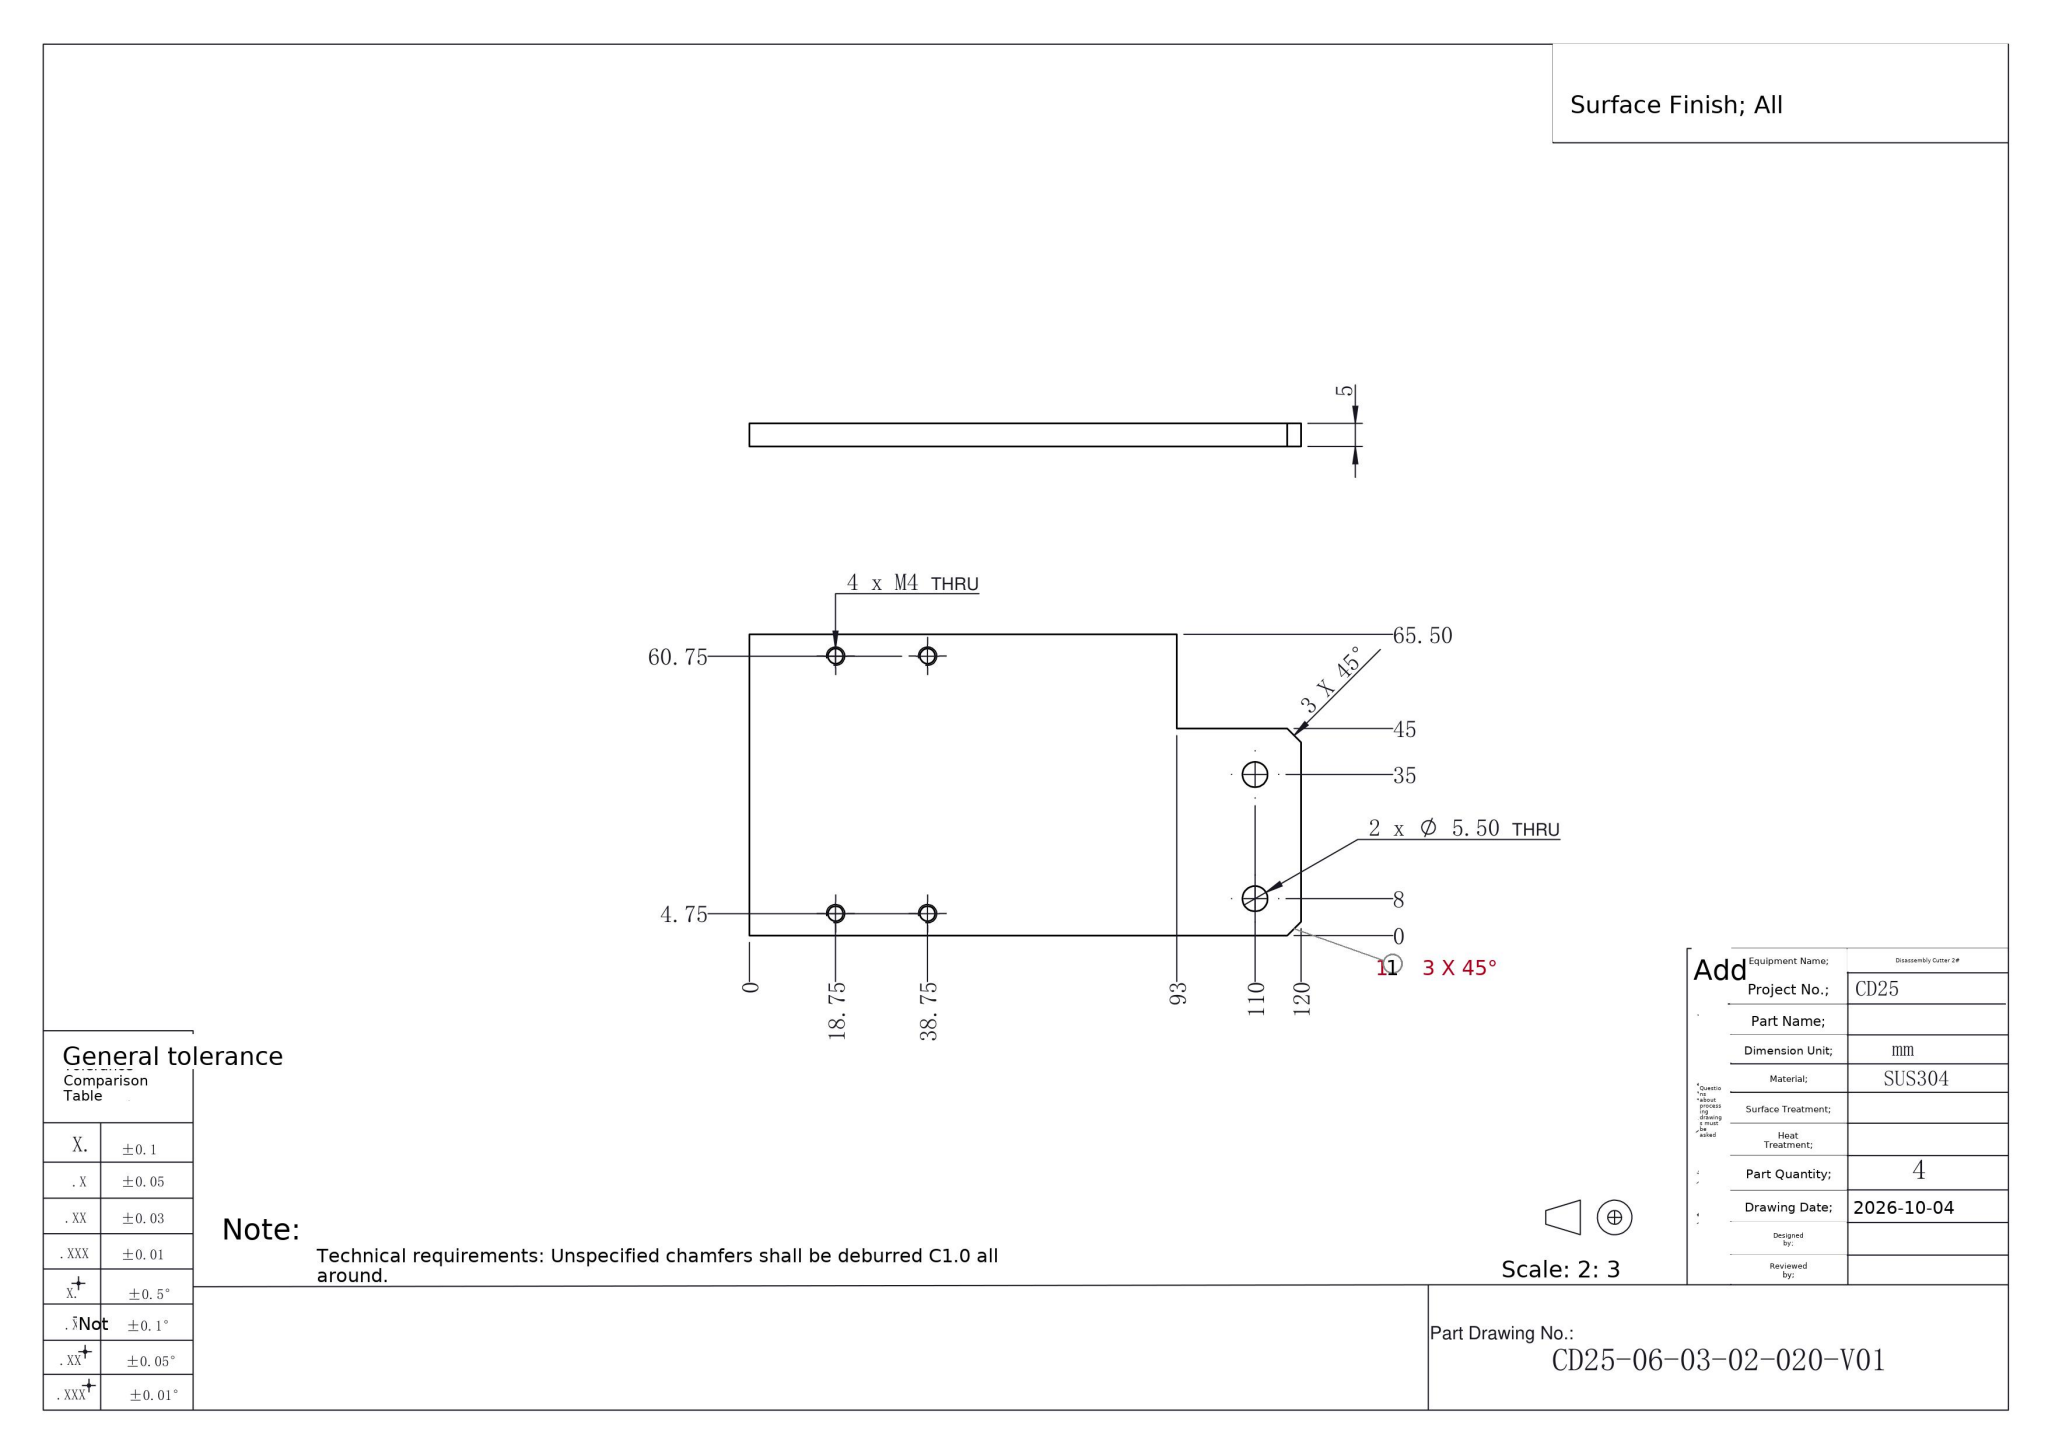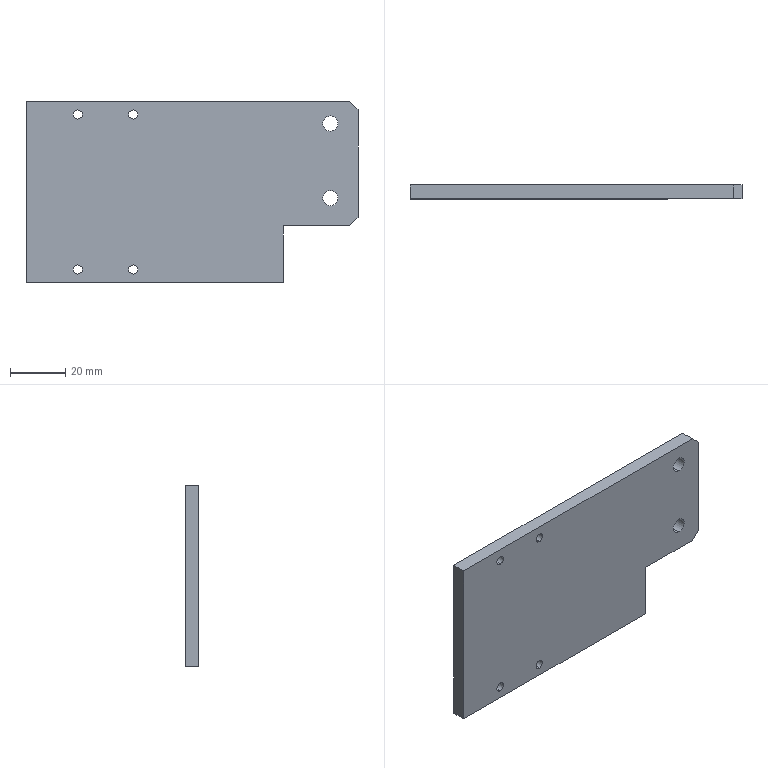Part | SolidWorks | mm | material SUS304 | 1 solid | 22 faces | box 120 x 5 x 65.5 mm | volume 36079 mm3 | cylinder 12 | plane 10 | commonest cylinder face diameters 3.3 x8 5.5 x4
build123d program:
from build123d import *

# Parameters (mm, degrees)
SKETCH1_W            = 120
SKETCH1_H            = 65.5
BOSS_EXTRUDE1_DEPTH  = 2.5
SKETCH2_W            = 27
SKETCH2_H            = 20.5
CUT_EXTRUDE1_DEPTH   = 69.539
CHAMFER1_SIZE        = 3
M5_CLEARANCE_HOLE1_D = 5.5
M4_TAPPED_HOLE1_D    = 3.3


with BuildPart() as part:
    # Sketch1 → Boss-Extrude1 (new, symmetric)
    with BuildSketch(Plane(origin=(0, 0, 0), x_dir=(1, 0, 0), z_dir=(0, 1, 0))):
        Rectangle(SKETCH1_W, SKETCH1_H)
    extrude(amount=BOSS_EXTRUDE1_DEPTH, both=True)

    # Sketch2 → Cut-Extrude1 (cut, through all)
    with BuildSketch(Plane(origin=(0, 2.5, 0), x_dir=(1, 0, 0), z_dir=(0, 1, 0))):
        with Locations((46.5, 22.5)):
            Rectangle(SKETCH2_W, SKETCH2_H)
    extrude(amount=-CUT_EXTRUDE1_DEPTH, mode=Mode.SUBTRACT)

    # Chamfer1
    chamfer1_edges = [part.edges().sort_by_distance(p)[0] for p in [
        (60, 0, -12.25),
        (60, 0, 32.75),
    ]]
    chamfer(chamfer1_edges, length=CHAMFER1_SIZE)

    # M5 Clearance Hole1 (through all)
    with Locations(Plane(origin=(0, 2.5, 0), x_dir=(1, 0, 0), z_dir=(0, 1, 0))):
        with Locations((50, 2.25), (50, -24.75)):
            Hole(M5_CLEARANCE_HOLE1_D / 2)

    # M4 Tapped Hole1 (through all)
    with Locations(Plane(origin=(0, 2.5, 0), x_dir=(1, 0, 0), z_dir=(0, 1, 0))):
        with Locations((-41.25, 28), (-21.25, 28), (-41.25, -28), (-21.25, -28)):
            Hole(M4_TAPPED_HOLE1_D / 2)


solid = part.part
STEP:
#1=CARTESIAN_POINT('',(-41.25,-2.5,-29.65));
#2=VERTEX_POINT('',#1);
#3=CARTESIAN_POINT('',(-41.25,-2.5,-26.35));
#4=VERTEX_POINT('',#3);
#5=CARTESIAN_POINT('',(-41.25,-2.5,-28.));
#6=DIRECTION('',(0.,1.,0.));
#7=DIRECTION('',(0.,0.,1.));
#8=AXIS2_PLACEMENT_3D('',#5,#6,#7);
#9=CIRCLE('',#8,1.65);
#10=EDGE_CURVE('',#2,#4,#9,.T.);
#11=ORIENTED_EDGE('',*,*,#10,.F.);
#12=CARTESIAN_POINT('',(-41.25,2.5,-29.65));
#13=VERTEX_POINT('',#12);
#14=CARTESIAN_POINT('',(-41.25,2.5,-29.65));
#15=DIRECTION('',(0.,1.,0.));
#16=VECTOR('',#15,1000.);
#17=LINE('',#14,#16);
#18=EDGE_CURVE('',#2,#13,#17,.T.);
#19=ORIENTED_EDGE('',*,*,#18,.T.);
#20=CARTESIAN_POINT('',(-41.25,2.5,-26.35));
#21=VERTEX_POINT('',#20);
#22=CARTESIAN_POINT('',(-41.25,2.5,-28.));
#23=DIRECTION('',(0.,1.,0.));
#24=DIRECTION('',(0.,0.,1.));
#25=AXIS2_PLACEMENT_3D('',#22,#23,#24);
#26=CIRCLE('',#25,1.65);
#27=EDGE_CURVE('',#13,#21,#26,.T.);
#28=ORIENTED_EDGE('',*,*,#27,.T.);
#29=CARTESIAN_POINT('',(-41.25,2.5,-26.35));
#30=DIRECTION('',(0.,1.,0.));
#31=VECTOR('',#30,1000.);
#32=LINE('',#29,#31);
#33=EDGE_CURVE('',#4,#21,#32,.T.);
#34=ORIENTED_EDGE('',*,*,#33,.F.);
#35=EDGE_LOOP('',(#11,#19,#28,#34));
#36=FACE_OUTER_BOUND('',#35,.T.);
#37=CARTESIAN_POINT('',(-41.25,2.5,-28.));
#38=DIRECTION('',(0.,1.,0.));
#39=DIRECTION('',(0.,0.,1.));
#40=AXIS2_PLACEMENT_3D('',#37,#38,#39);
#41=CYLINDRICAL_SURFACE('',#40,1.65);
#42=ADVANCED_FACE('',(#36),#41,.F.);
#43=CARTESIAN_POINT('',(-21.25,-2.5,-29.65));
#44=VERTEX_POINT('',#43);
#45=CARTESIAN_POINT('',(-21.25,-2.5,-26.35));
#46=VERTEX_POINT('',#45);
#47=CARTESIAN_POINT('',(-21.25,-2.5,-28.));
#48=DIRECTION('',(0.,1.,0.));
#49=DIRECTION('',(0.,0.,1.));
#50=AXIS2_PLACEMENT_3D('',#47,#48,#49);
#51=CIRCLE('',#50,1.65);
#52=EDGE_CURVE('',#44,#46,#51,.T.);
#53=ORIENTED_EDGE('',*,*,#52,.F.);
#54=CARTESIAN_POINT('',(-21.25,2.5,-29.65));
#55=VERTEX_POINT('',#54);
#56=CARTESIAN_POINT('',(-21.25,2.5,-29.65));
#57=DIRECTION('',(0.,1.,0.));
#58=VECTOR('',#57,1000.);
#59=LINE('',#56,#58);
#60=EDGE_CURVE('',#44,#55,#59,.T.);
#61=ORIENTED_EDGE('',*,*,#60,.T.);
#62=CARTESIAN_POINT('',(-21.25,2.5,-26.35));
#63=VERTEX_POINT('',#62);
#64=CARTESIAN_POINT('',(-21.25,2.5,-28.));
#65=DIRECTION('',(0.,1.,0.));
#66=DIRECTION('',(0.,0.,1.));
#67=AXIS2_PLACEMENT_3D('',#64,#65,#66);
#68=CIRCLE('',#67,1.65);
#69=EDGE_CURVE('',#55,#63,#68,.T.);
#70=ORIENTED_EDGE('',*,*,#69,.T.);
#71=CARTESIAN_POINT('',(-21.25,2.5,-26.35));
#72=DIRECTION('',(0.,1.,0.));
#73=VECTOR('',#72,1000.);
#74=LINE('',#71,#73);
#75=EDGE_CURVE('',#46,#63,#74,.T.);
#76=ORIENTED_EDGE('',*,*,#75,.F.);
#77=EDGE_LOOP('',(#53,#61,#70,#76));
#78=FACE_OUTER_BOUND('',#77,.T.);
#79=CARTESIAN_POINT('',(-21.25,2.5,-28.));
#80=DIRECTION('',(0.,1.,0.));
#81=DIRECTION('',(0.,0.,1.));
#82=AXIS2_PLACEMENT_3D('',#79,#80,#81);
#83=CYLINDRICAL_SURFACE('',#82,1.65);
#84=ADVANCED_FACE('',(#78),#83,.F.);
#85=CARTESIAN_POINT('',(-41.25,-2.5,26.35));
#86=VERTEX_POINT('',#85);
#87=CARTESIAN_POINT('',(-41.25,-2.5,29.65));
#88=VERTEX_POINT('',#87);
#89=CARTESIAN_POINT('',(-41.25,-2.5,28.));
#90=DIRECTION('',(0.,1.,0.));
#91=DIRECTION('',(0.,0.,1.));
#92=AXIS2_PLACEMENT_3D('',#89,#90,#91);
#93=CIRCLE('',#92,1.65);
#94=EDGE_CURVE('',#86,#88,#93,.T.);
#95=ORIENTED_EDGE('',*,*,#94,.F.);
#96=CARTESIAN_POINT('',(-41.25,2.5,26.35));
#97=VERTEX_POINT('',#96);
#98=CARTESIAN_POINT('',(-41.25,2.5,26.35));
#99=DIRECTION('',(0.,1.,0.));
#100=VECTOR('',#99,1000.);
#101=LINE('',#98,#100);
#102=EDGE_CURVE('',#86,#97,#101,.T.);
#103=ORIENTED_EDGE('',*,*,#102,.T.);
#104=CARTESIAN_POINT('',(-41.25,2.5,29.65));
#105=VERTEX_POINT('',#104);
#106=CARTESIAN_POINT('',(-41.25,2.5,28.));
#107=DIRECTION('',(0.,1.,0.));
#108=DIRECTION('',(0.,0.,1.));
#109=AXIS2_PLACEMENT_3D('',#106,#107,#108);
#110=CIRCLE('',#109,1.65);
#111=EDGE_CURVE('',#97,#105,#110,.T.);
#112=ORIENTED_EDGE('',*,*,#111,.T.);
#113=CARTESIAN_POINT('',(-41.25,2.5,29.65));
#114=DIRECTION('',(0.,1.,0.));
#115=VECTOR('',#114,1000.);
#116=LINE('',#113,#115);
#117=EDGE_CURVE('',#88,#105,#116,.T.);
#118=ORIENTED_EDGE('',*,*,#117,.F.);
#119=EDGE_LOOP('',(#95,#103,#112,#118));
#120=FACE_OUTER_BOUND('',#119,.T.);
#121=CARTESIAN_POINT('',(-41.25,2.5,28.));
#122=DIRECTION('',(0.,1.,0.));
#123=DIRECTION('',(0.,0.,1.));
#124=AXIS2_PLACEMENT_3D('',#121,#122,#123);
#125=CYLINDRICAL_SURFACE('',#124,1.65);
#126=ADVANCED_FACE('',(#120),#125,.F.);
#127=CARTESIAN_POINT('',(-21.25,-2.5,26.35));
#128=VERTEX_POINT('',#127);
#129=CARTESIAN_POINT('',(-21.25,-2.5,29.65));
#130=VERTEX_POINT('',#129);
#131=CARTESIAN_POINT('',(-21.25,-2.5,28.));
#132=DIRECTION('',(0.,1.,0.));
#133=DIRECTION('',(0.,0.,1.));
#134=AXIS2_PLACEMENT_3D('',#131,#132,#133);
#135=CIRCLE('',#134,1.65);
#136=EDGE_CURVE('',#128,#130,#135,.T.);
#137=ORIENTED_EDGE('',*,*,#136,.F.);
#138=CARTESIAN_POINT('',(-21.25,2.5,26.35));
#139=VERTEX_POINT('',#138);
#140=CARTESIAN_POINT('',(-21.25,2.5,26.35));
#141=DIRECTION('',(0.,1.,0.));
#142=VECTOR('',#141,1000.);
#143=LINE('',#140,#142);
#144=EDGE_CURVE('',#128,#139,#143,.T.);
#145=ORIENTED_EDGE('',*,*,#144,.T.);
#146=CARTESIAN_POINT('',(-21.25,2.5,29.65));
#147=VERTEX_POINT('',#146);
#148=CARTESIAN_POINT('',(-21.25,2.5,28.));
#149=DIRECTION('',(0.,1.,0.));
#150=DIRECTION('',(0.,0.,1.));
#151=AXIS2_PLACEMENT_3D('',#148,#149,#150);
#152=CIRCLE('',#151,1.65);
#153=EDGE_CURVE('',#139,#147,#152,.T.);
#154=ORIENTED_EDGE('',*,*,#153,.T.);
#155=CARTESIAN_POINT('',(-21.25,2.5,29.65));
#156=DIRECTION('',(0.,1.,0.));
#157=VECTOR('',#156,1000.);
#158=LINE('',#155,#157);
#159=EDGE_CURVE('',#130,#147,#158,.T.);
#160=ORIENTED_EDGE('',*,*,#159,.F.);
#161=EDGE_LOOP('',(#137,#145,#154,#160));
#162=FACE_OUTER_BOUND('',#161,.T.);
#163=CARTESIAN_POINT('',(-21.25,2.5,28.));
#164=DIRECTION('',(0.,1.,0.));
#165=DIRECTION('',(0.,0.,1.));
#166=AXIS2_PLACEMENT_3D('',#163,#164,#165);
#167=CYLINDRICAL_SURFACE('',#166,1.65);
#168=ADVANCED_FACE('',(#162),#167,.F.);
#169=CARTESIAN_POINT('',(50.,-2.5,-5.));
#170=VERTEX_POINT('',#169);
#171=CARTESIAN_POINT('',(50.,-2.5,0.5));
#172=VERTEX_POINT('',#171);
#173=CARTESIAN_POINT('',(50.,-2.5,-2.25));
#174=DIRECTION('',(0.,1.,0.));
#175=DIRECTION('',(0.,0.,1.));
#176=AXIS2_PLACEMENT_3D('',#173,#174,#175);
#177=CIRCLE('',#176,2.75);
#178=EDGE_CURVE('',#170,#172,#177,.T.);
#179=ORIENTED_EDGE('',*,*,#178,.F.);
#180=CARTESIAN_POINT('',(50.,2.5,-5.));
#181=VERTEX_POINT('',#180);
#182=CARTESIAN_POINT('',(50.,2.5,-5.));
#183=DIRECTION('',(0.,1.,0.));
#184=VECTOR('',#183,1000.);
#185=LINE('',#182,#184);
#186=EDGE_CURVE('',#170,#181,#185,.T.);
#187=ORIENTED_EDGE('',*,*,#186,.T.);
#188=CARTESIAN_POINT('',(50.,2.5,0.5));
#189=VERTEX_POINT('',#188);
#190=CARTESIAN_POINT('',(50.,2.5,-2.25));
#191=DIRECTION('',(0.,1.,0.));
#192=DIRECTION('',(0.,0.,1.));
#193=AXIS2_PLACEMENT_3D('',#190,#191,#192);
#194=CIRCLE('',#193,2.75);
#195=EDGE_CURVE('',#181,#189,#194,.T.);
#196=ORIENTED_EDGE('',*,*,#195,.T.);
#197=CARTESIAN_POINT('',(50.,2.5,0.5));
#198=DIRECTION('',(0.,1.,0.));
#199=VECTOR('',#198,1000.);
#200=LINE('',#197,#199);
#201=EDGE_CURVE('',#172,#189,#200,.T.);
#202=ORIENTED_EDGE('',*,*,#201,.F.);
#203=EDGE_LOOP('',(#179,#187,#196,#202));
#204=FACE_OUTER_BOUND('',#203,.T.);
#205=CARTESIAN_POINT('',(50.,2.5,-2.25));
#206=DIRECTION('',(0.,1.,0.));
#207=DIRECTION('',(0.,0.,1.));
#208=AXIS2_PLACEMENT_3D('',#205,#206,#207);
#209=CYLINDRICAL_SURFACE('',#208,2.75);
#210=ADVANCED_FACE('',(#204),#209,.F.);
#211=CARTESIAN_POINT('',(50.,-2.5,22.));
#212=VERTEX_POINT('',#211);
#213=CARTESIAN_POINT('',(50.,-2.5,27.5));
#214=VERTEX_POINT('',#213);
#215=CARTESIAN_POINT('',(50.,-2.5,24.75));
#216=DIRECTION('',(0.,1.,0.));
#217=DIRECTION('',(0.,0.,1.));
#218=AXIS2_PLACEMENT_3D('',#215,#216,#217);
#219=CIRCLE('',#218,2.75);
#220=EDGE_CURVE('',#212,#214,#219,.T.);
#221=ORIENTED_EDGE('',*,*,#220,.F.);
#222=CARTESIAN_POINT('',(50.,2.5,22.));
#223=VERTEX_POINT('',#222);
#224=CARTESIAN_POINT('',(50.,2.5,22.));
#225=DIRECTION('',(0.,1.,0.));
#226=VECTOR('',#225,1000.);
#227=LINE('',#224,#226);
#228=EDGE_CURVE('',#212,#223,#227,.T.);
#229=ORIENTED_EDGE('',*,*,#228,.T.);
#230=CARTESIAN_POINT('',(50.,2.5,27.5));
#231=VERTEX_POINT('',#230);
#232=CARTESIAN_POINT('',(50.,2.5,24.75));
#233=DIRECTION('',(0.,1.,0.));
#234=DIRECTION('',(0.,0.,1.));
#235=AXIS2_PLACEMENT_3D('',#232,#233,#234);
#236=CIRCLE('',#235,2.75);
#237=EDGE_CURVE('',#223,#231,#236,.T.);
#238=ORIENTED_EDGE('',*,*,#237,.T.);
#239=CARTESIAN_POINT('',(50.,2.5,27.5));
#240=DIRECTION('',(0.,1.,0.));
#241=VECTOR('',#240,1000.);
#242=LINE('',#239,#241);
#243=EDGE_CURVE('',#214,#231,#242,.T.);
#244=ORIENTED_EDGE('',*,*,#243,.F.);
#245=EDGE_LOOP('',(#221,#229,#238,#244));
#246=FACE_OUTER_BOUND('',#245,.T.);
#247=CARTESIAN_POINT('',(50.,2.5,24.75));
#248=DIRECTION('',(0.,1.,0.));
#249=DIRECTION('',(0.,0.,1.));
#250=AXIS2_PLACEMENT_3D('',#247,#248,#249);
#251=CYLINDRICAL_SURFACE('',#250,2.75);
#252=ADVANCED_FACE('',(#246),#251,.F.);
#253=CARTESIAN_POINT('',(60.,-2.5,29.75));
#254=VERTEX_POINT('',#253);
#255=CARTESIAN_POINT('',(60.,-2.5,-9.25));
#256=VERTEX_POINT('',#255);
#257=CARTESIAN_POINT('',(60.,-2.5,-32.75));
#258=DIRECTION('',(-0.,0.,-1.));
#259=VECTOR('',#258,1000.);
#260=LINE('',#257,#259);
#261=EDGE_CURVE('',#254,#256,#260,.T.);
#262=ORIENTED_EDGE('',*,*,#261,.T.);
#263=CARTESIAN_POINT('',(60.,2.5,-9.25));
#264=VERTEX_POINT('',#263);
#265=CARTESIAN_POINT('',(60.,2.5,-9.25));
#266=DIRECTION('',(0.,1.,0.));
#267=VECTOR('',#266,1000.);
#268=LINE('',#265,#267);
#269=EDGE_CURVE('',#256,#264,#268,.T.);
#270=ORIENTED_EDGE('',*,*,#269,.T.);
#271=CARTESIAN_POINT('',(60.,2.5,29.75));
#272=VERTEX_POINT('',#271);
#273=CARTESIAN_POINT('',(60.,2.5,-32.75));
#274=DIRECTION('',(-0.,0.,-1.));
#275=VECTOR('',#274,1000.);
#276=LINE('',#273,#275);
#277=EDGE_CURVE('',#272,#264,#276,.T.);
#278=ORIENTED_EDGE('',*,*,#277,.F.);
#279=CARTESIAN_POINT('',(60.,2.5,29.75));
#280=DIRECTION('',(0.,-1.,0.));
#281=VECTOR('',#280,1000.);
#282=LINE('',#279,#281);
#283=EDGE_CURVE('',#272,#254,#282,.T.);
#284=ORIENTED_EDGE('',*,*,#283,.T.);
#285=EDGE_LOOP('',(#262,#270,#278,#284));
#286=FACE_OUTER_BOUND('',#285,.T.);
#287=CARTESIAN_POINT('',(60.,2.5,-32.75));
#288=DIRECTION('',(-1.,0.,0.));
#289=DIRECTION('',(0.,0.,1.));
#290=AXIS2_PLACEMENT_3D('',#287,#288,#289);
#291=PLANE('',#290);
#292=ADVANCED_FACE('',(#286),#291,.F.);
#293=CARTESIAN_POINT('',(33.,2.5,-32.75));
#294=VERTEX_POINT('',#293);
#295=CARTESIAN_POINT('',(-60.,2.5,-32.75));
#296=VERTEX_POINT('',#295);
#297=CARTESIAN_POINT('',(-60.,2.5,-32.75));
#298=DIRECTION('',(-1.,0.,0.));
#299=VECTOR('',#298,1000.);
#300=LINE('',#297,#299);
#301=EDGE_CURVE('',#294,#296,#300,.T.);
#302=ORIENTED_EDGE('',*,*,#301,.F.);
#303=CARTESIAN_POINT('',(33.,-2.5,-32.75));
#304=VERTEX_POINT('',#303);
#305=CARTESIAN_POINT('',(33.,-2.5,-32.75));
#306=DIRECTION('',(0.,1.,0.));
#307=VECTOR('',#306,1000.);
#308=LINE('',#305,#307);
#309=EDGE_CURVE('',#304,#294,#308,.T.);
#310=ORIENTED_EDGE('',*,*,#309,.F.);
#311=CARTESIAN_POINT('',(-60.,-2.5,-32.75));
#312=VERTEX_POINT('',#311);
#313=CARTESIAN_POINT('',(-60.,-2.5,-32.75));
#314=DIRECTION('',(-1.,0.,0.));
#315=VECTOR('',#314,1000.);
#316=LINE('',#313,#315);
#317=EDGE_CURVE('',#304,#312,#316,.T.);
#318=ORIENTED_EDGE('',*,*,#317,.T.);
#319=CARTESIAN_POINT('',(-60.,2.5,-32.75));
#320=DIRECTION('',(0.,-1.,0.));
#321=VECTOR('',#320,1000.);
#322=LINE('',#319,#321);
#323=EDGE_CURVE('',#296,#312,#322,.T.);
#324=ORIENTED_EDGE('',*,*,#323,.F.);
#325=EDGE_LOOP('',(#302,#310,#318,#324));
#326=FACE_OUTER_BOUND('',#325,.T.);
#327=CARTESIAN_POINT('',(-60.,2.5,-32.75));
#328=DIRECTION('',(0.,0.,1.));
#329=DIRECTION('',(1.,0.,0.));
#330=AXIS2_PLACEMENT_3D('',#327,#328,#329);
#331=PLANE('',#330);
#332=ADVANCED_FACE('',(#326),#331,.F.);
#333=CARTESIAN_POINT('',(-60.,-2.5,32.75));
#334=VERTEX_POINT('',#333);
#335=CARTESIAN_POINT('',(-60.,-2.5,-32.75));
#336=DIRECTION('',(0.,0.,1.));
#337=VECTOR('',#336,1000.);
#338=LINE('',#335,#337);
#339=EDGE_CURVE('',#312,#334,#338,.T.);
#340=ORIENTED_EDGE('',*,*,#339,.T.);
#341=CARTESIAN_POINT('',(-60.,2.5,32.75));
#342=VERTEX_POINT('',#341);
#343=CARTESIAN_POINT('',(-60.,2.5,32.75));
#344=DIRECTION('',(0.,-1.,0.));
#345=VECTOR('',#344,1000.);
#346=LINE('',#343,#345);
#347=EDGE_CURVE('',#342,#334,#346,.T.);
#348=ORIENTED_EDGE('',*,*,#347,.F.);
#349=CARTESIAN_POINT('',(-60.,2.5,-32.75));
#350=DIRECTION('',(0.,0.,1.));
#351=VECTOR('',#350,1000.);
#352=LINE('',#349,#351);
#353=EDGE_CURVE('',#296,#342,#352,.T.);
#354=ORIENTED_EDGE('',*,*,#353,.F.);
#355=ORIENTED_EDGE('',*,*,#323,.T.);
#356=EDGE_LOOP('',(#340,#348,#354,#355));
#357=FACE_OUTER_BOUND('',#356,.T.);
#358=CARTESIAN_POINT('',(-60.,2.5,-32.75));
#359=DIRECTION('',(1.,0.,-0.));
#360=DIRECTION('',(-0.,0.,-1.));
#361=AXIS2_PLACEMENT_3D('',#358,#359,#360);
#362=PLANE('',#361);
#363=ADVANCED_FACE('',(#357),#362,.F.);
#364=CARTESIAN_POINT('',(57.,-2.5,32.75));
#365=VERTEX_POINT('',#364);
#366=CARTESIAN_POINT('',(-60.,-2.5,32.75));
#367=DIRECTION('',(1.,0.,0.));
#368=VECTOR('',#367,1000.);
#369=LINE('',#366,#368);
#370=EDGE_CURVE('',#334,#365,#369,.T.);
#371=ORIENTED_EDGE('',*,*,#370,.T.);
#372=CARTESIAN_POINT('',(57.,2.5,32.75));
#373=VERTEX_POINT('',#372);
#374=CARTESIAN_POINT('',(57.,2.5,32.75));
#375=DIRECTION('',(0.,1.,0.));
#376=VECTOR('',#375,1000.);
#377=LINE('',#374,#376);
#378=EDGE_CURVE('',#365,#373,#377,.T.);
#379=ORIENTED_EDGE('',*,*,#378,.T.);
#380=CARTESIAN_POINT('',(-60.,2.5,32.75));
#381=DIRECTION('',(1.,0.,0.));
#382=VECTOR('',#381,1000.);
#383=LINE('',#380,#382);
#384=EDGE_CURVE('',#342,#373,#383,.T.);
#385=ORIENTED_EDGE('',*,*,#384,.F.);
#386=ORIENTED_EDGE('',*,*,#347,.T.);
#387=EDGE_LOOP('',(#371,#379,#385,#386));
#388=FACE_OUTER_BOUND('',#387,.T.);
#389=CARTESIAN_POINT('',(-60.,2.5,32.75));
#390=DIRECTION('',(0.,0.,-1.));
#391=DIRECTION('',(-1.,0.,0.));
#392=AXIS2_PLACEMENT_3D('',#389,#390,#391);
#393=PLANE('',#392);
#394=ADVANCED_FACE('',(#388),#393,.F.);
#395=CARTESIAN_POINT('',(-41.25,2.5,-28.));
#396=DIRECTION('',(0.,1.,0.));
#397=DIRECTION('',(0.,0.,1.));
#398=AXIS2_PLACEMENT_3D('',#395,#396,#397);
#399=CIRCLE('',#398,1.65);
#400=EDGE_CURVE('',#21,#13,#399,.T.);
#401=ORIENTED_EDGE('',*,*,#400,.F.);
#402=ORIENTED_EDGE('',*,*,#27,.F.);
#403=EDGE_LOOP('',(#401,#402));
#404=FACE_BOUND('',#403,.T.);
#405=CARTESIAN_POINT('',(-21.25,2.5,-28.));
#406=DIRECTION('',(0.,1.,0.));
#407=DIRECTION('',(0.,0.,1.));
#408=AXIS2_PLACEMENT_3D('',#405,#406,#407);
#409=CIRCLE('',#408,1.65);
#410=EDGE_CURVE('',#63,#55,#409,.T.);
#411=ORIENTED_EDGE('',*,*,#410,.F.);
#412=ORIENTED_EDGE('',*,*,#69,.F.);
#413=EDGE_LOOP('',(#411,#412));
#414=FACE_BOUND('',#413,.T.);
#415=CARTESIAN_POINT('',(-41.25,2.5,28.));
#416=DIRECTION('',(0.,1.,0.));
#417=DIRECTION('',(0.,0.,1.));
#418=AXIS2_PLACEMENT_3D('',#415,#416,#417);
#419=CIRCLE('',#418,1.65);
#420=EDGE_CURVE('',#105,#97,#419,.T.);
#421=ORIENTED_EDGE('',*,*,#420,.F.);
#422=ORIENTED_EDGE('',*,*,#111,.F.);
#423=EDGE_LOOP('',(#421,#422));
#424=FACE_BOUND('',#423,.T.);
#425=CARTESIAN_POINT('',(-21.25,2.5,28.));
#426=DIRECTION('',(0.,1.,0.));
#427=DIRECTION('',(0.,0.,1.));
#428=AXIS2_PLACEMENT_3D('',#425,#426,#427);
#429=CIRCLE('',#428,1.65);
#430=EDGE_CURVE('',#147,#139,#429,.T.);
#431=ORIENTED_EDGE('',*,*,#430,.F.);
#432=ORIENTED_EDGE('',*,*,#153,.F.);
#433=EDGE_LOOP('',(#431,#432));
#434=FACE_BOUND('',#433,.T.);
#435=CARTESIAN_POINT('',(50.,2.5,-2.25));
#436=DIRECTION('',(0.,1.,0.));
#437=DIRECTION('',(0.,0.,1.));
#438=AXIS2_PLACEMENT_3D('',#435,#436,#437);
#439=CIRCLE('',#438,2.75);
#440=EDGE_CURVE('',#189,#181,#439,.T.);
#441=ORIENTED_EDGE('',*,*,#440,.F.);
#442=ORIENTED_EDGE('',*,*,#195,.F.);
#443=EDGE_LOOP('',(#441,#442));
#444=FACE_BOUND('',#443,.T.);
#445=CARTESIAN_POINT('',(50.,2.5,24.75));
#446=DIRECTION('',(0.,1.,0.));
#447=DIRECTION('',(0.,0.,1.));
#448=AXIS2_PLACEMENT_3D('',#445,#446,#447);
#449=CIRCLE('',#448,2.75);
#450=EDGE_CURVE('',#231,#223,#449,.T.);
#451=ORIENTED_EDGE('',*,*,#450,.F.);
#452=ORIENTED_EDGE('',*,*,#237,.F.);
#453=EDGE_LOOP('',(#451,#452));
#454=FACE_BOUND('',#453,.T.);
#455=ORIENTED_EDGE('',*,*,#277,.T.);
#456=CARTESIAN_POINT('',(57.,2.5,-12.25));
#457=VERTEX_POINT('',#456);
#458=CARTESIAN_POINT('',(34.625,2.5,-34.625));
#459=DIRECTION('',(-0.7071,0.,-0.7071));
#460=VECTOR('',#459,1000.);
#461=LINE('',#458,#460);
#462=EDGE_CURVE('',#264,#457,#461,.T.);
#463=ORIENTED_EDGE('',*,*,#462,.T.);
#464=CARTESIAN_POINT('',(33.,2.5,-12.25));
#465=VERTEX_POINT('',#464);
#466=CARTESIAN_POINT('',(60.,2.5,-12.25));
#467=DIRECTION('',(1.,0.,-0.));
#468=VECTOR('',#467,1000.);
#469=LINE('',#466,#468);
#470=EDGE_CURVE('',#465,#457,#469,.T.);
#471=ORIENTED_EDGE('',*,*,#470,.F.);
#472=CARTESIAN_POINT('',(33.,2.5,-32.75));
#473=DIRECTION('',(0.,0.,1.));
#474=VECTOR('',#473,1000.);
#475=LINE('',#472,#474);
#476=EDGE_CURVE('',#294,#465,#475,.T.);
#477=ORIENTED_EDGE('',*,*,#476,.F.);
#478=ORIENTED_EDGE('',*,*,#301,.T.);
#479=ORIENTED_EDGE('',*,*,#353,.T.);
#480=ORIENTED_EDGE('',*,*,#384,.T.);
#481=CARTESIAN_POINT('',(44.875,2.5,44.875));
#482=DIRECTION('',(0.7071,0.,-0.7071));
#483=VECTOR('',#482,1000.);
#484=LINE('',#481,#483);
#485=EDGE_CURVE('',#373,#272,#484,.T.);
#486=ORIENTED_EDGE('',*,*,#485,.T.);
#487=EDGE_LOOP('',(#455,#463,#471,#477,#478,#479,#480,#486));
#488=FACE_OUTER_BOUND('',#487,.T.);
#489=CARTESIAN_POINT('',(0.,2.5,0.));
#490=DIRECTION('',(0.,1.,0.));
#491=DIRECTION('',(0.,0.,1.));
#492=AXIS2_PLACEMENT_3D('',#489,#490,#491);
#493=PLANE('',#492);
#494=ADVANCED_FACE('',(#404,#414,#424,#434,#444,#454,#488),#493,.T.);
#495=CARTESIAN_POINT('',(-41.25,-2.5,-28.));
#496=DIRECTION('',(0.,1.,0.));
#497=DIRECTION('',(0.,0.,1.));
#498=AXIS2_PLACEMENT_3D('',#495,#496,#497);
#499=CIRCLE('',#498,1.65);
#500=EDGE_CURVE('',#4,#2,#499,.T.);
#501=ORIENTED_EDGE('',*,*,#500,.T.);
#502=ORIENTED_EDGE('',*,*,#10,.T.);
#503=EDGE_LOOP('',(#501,#502));
#504=FACE_BOUND('',#503,.T.);
#505=CARTESIAN_POINT('',(-21.25,-2.5,-28.));
#506=DIRECTION('',(0.,1.,0.));
#507=DIRECTION('',(0.,0.,1.));
#508=AXIS2_PLACEMENT_3D('',#505,#506,#507);
#509=CIRCLE('',#508,1.65);
#510=EDGE_CURVE('',#46,#44,#509,.T.);
#511=ORIENTED_EDGE('',*,*,#510,.T.);
#512=ORIENTED_EDGE('',*,*,#52,.T.);
#513=EDGE_LOOP('',(#511,#512));
#514=FACE_BOUND('',#513,.T.);
#515=CARTESIAN_POINT('',(-41.25,-2.5,28.));
#516=DIRECTION('',(0.,1.,0.));
#517=DIRECTION('',(0.,0.,1.));
#518=AXIS2_PLACEMENT_3D('',#515,#516,#517);
#519=CIRCLE('',#518,1.65);
#520=EDGE_CURVE('',#88,#86,#519,.T.);
#521=ORIENTED_EDGE('',*,*,#520,.T.);
#522=ORIENTED_EDGE('',*,*,#94,.T.);
#523=EDGE_LOOP('',(#521,#522));
#524=FACE_BOUND('',#523,.T.);
#525=CARTESIAN_POINT('',(-21.25,-2.5,28.));
#526=DIRECTION('',(0.,1.,0.));
#527=DIRECTION('',(0.,0.,1.));
#528=AXIS2_PLACEMENT_3D('',#525,#526,#527);
#529=CIRCLE('',#528,1.65);
#530=EDGE_CURVE('',#130,#128,#529,.T.);
#531=ORIENTED_EDGE('',*,*,#530,.T.);
#532=ORIENTED_EDGE('',*,*,#136,.T.);
#533=EDGE_LOOP('',(#531,#532));
#534=FACE_BOUND('',#533,.T.);
#535=CARTESIAN_POINT('',(50.,-2.5,-2.25));
#536=DIRECTION('',(0.,1.,0.));
#537=DIRECTION('',(0.,0.,1.));
#538=AXIS2_PLACEMENT_3D('',#535,#536,#537);
#539=CIRCLE('',#538,2.75);
#540=EDGE_CURVE('',#172,#170,#539,.T.);
#541=ORIENTED_EDGE('',*,*,#540,.T.);
#542=ORIENTED_EDGE('',*,*,#178,.T.);
#543=EDGE_LOOP('',(#541,#542));
#544=FACE_BOUND('',#543,.T.);
#545=CARTESIAN_POINT('',(50.,-2.5,24.75));
#546=DIRECTION('',(0.,1.,0.));
#547=DIRECTION('',(0.,0.,1.));
#548=AXIS2_PLACEMENT_3D('',#545,#546,#547);
#549=CIRCLE('',#548,2.75);
#550=EDGE_CURVE('',#214,#212,#549,.T.);
#551=ORIENTED_EDGE('',*,*,#550,.T.);
#552=ORIENTED_EDGE('',*,*,#220,.T.);
#553=EDGE_LOOP('',(#551,#552));
#554=FACE_BOUND('',#553,.T.);
#555=CARTESIAN_POINT('',(33.,-2.5,-12.25));
#556=VERTEX_POINT('',#555);
#557=CARTESIAN_POINT('',(57.,-2.5,-12.25));
#558=VERTEX_POINT('',#557);
#559=CARTESIAN_POINT('',(60.,-2.5,-12.25));
#560=DIRECTION('',(1.,0.,-0.));
#561=VECTOR('',#560,1000.);
#562=LINE('',#559,#561);
#563=EDGE_CURVE('',#556,#558,#562,.T.);
#564=ORIENTED_EDGE('',*,*,#563,.T.);
#565=CARTESIAN_POINT('',(60.,-2.5,-9.25));
#566=DIRECTION('',(0.7071,0.,0.7071));
#567=VECTOR('',#566,1000.);
#568=LINE('',#565,#567);
#569=EDGE_CURVE('',#558,#256,#568,.T.);
#570=ORIENTED_EDGE('',*,*,#569,.T.);
#571=ORIENTED_EDGE('',*,*,#261,.F.);
#572=CARTESIAN_POINT('',(60.,-2.5,29.75));
#573=DIRECTION('',(-0.7071,0.,0.7071));
#574=VECTOR('',#573,1000.);
#575=LINE('',#572,#574);
#576=EDGE_CURVE('',#254,#365,#575,.T.);
#577=ORIENTED_EDGE('',*,*,#576,.T.);
#578=ORIENTED_EDGE('',*,*,#370,.F.);
#579=ORIENTED_EDGE('',*,*,#339,.F.);
#580=ORIENTED_EDGE('',*,*,#317,.F.);
#581=CARTESIAN_POINT('',(33.,-2.5,-32.75));
#582=DIRECTION('',(0.,0.,1.));
#583=VECTOR('',#582,1000.);
#584=LINE('',#581,#583);
#585=EDGE_CURVE('',#304,#556,#584,.T.);
#586=ORIENTED_EDGE('',*,*,#585,.T.);
#587=EDGE_LOOP('',(#564,#570,#571,#577,#578,#579,#580,#586));
#588=FACE_OUTER_BOUND('',#587,.T.);
#589=CARTESIAN_POINT('',(0.,-2.5,0.));
#590=DIRECTION('',(0.,1.,0.));
#591=DIRECTION('',(0.,0.,1.));
#592=AXIS2_PLACEMENT_3D('',#589,#590,#591);
#593=PLANE('',#592);
#594=ADVANCED_FACE('',(#504,#514,#524,#534,#544,#554,#588),#593,.F.);
#595=ORIENTED_EDGE('',*,*,#470,.T.);
#596=CARTESIAN_POINT('',(57.,-2.5,-12.25));
#597=DIRECTION('',(0.,-1.,0.));
#598=VECTOR('',#597,1000.);
#599=LINE('',#596,#598);
#600=EDGE_CURVE('',#457,#558,#599,.T.);
#601=ORIENTED_EDGE('',*,*,#600,.T.);
#602=ORIENTED_EDGE('',*,*,#563,.F.);
#603=CARTESIAN_POINT('',(33.,-2.5,-12.25));
#604=DIRECTION('',(0.,1.,0.));
#605=VECTOR('',#604,1000.);
#606=LINE('',#603,#605);
#607=EDGE_CURVE('',#556,#465,#606,.T.);
#608=ORIENTED_EDGE('',*,*,#607,.T.);
#609=EDGE_LOOP('',(#595,#601,#602,#608));
#610=FACE_OUTER_BOUND('',#609,.T.);
#611=CARTESIAN_POINT('',(60.,-2.5,-12.25));
#612=DIRECTION('',(0.,0.,1.));
#613=DIRECTION('',(1.,0.,-0.));
#614=AXIS2_PLACEMENT_3D('',#611,#612,#613);
#615=PLANE('',#614);
#616=ADVANCED_FACE('',(#610),#615,.F.);
#617=ORIENTED_EDGE('',*,*,#476,.T.);
#618=ORIENTED_EDGE('',*,*,#607,.F.);
#619=ORIENTED_EDGE('',*,*,#585,.F.);
#620=ORIENTED_EDGE('',*,*,#309,.T.);
#621=EDGE_LOOP('',(#617,#618,#619,#620));
#622=FACE_OUTER_BOUND('',#621,.T.);
#623=CARTESIAN_POINT('',(33.,-2.5,-32.75));
#624=DIRECTION('',(-1.,0.,0.));
#625=DIRECTION('',(0.,0.,1.));
#626=AXIS2_PLACEMENT_3D('',#623,#624,#625);
#627=PLANE('',#626);
#628=ADVANCED_FACE('',(#622),#627,.F.);
#629=ORIENTED_EDGE('',*,*,#569,.F.);
#630=ORIENTED_EDGE('',*,*,#600,.F.);
#631=ORIENTED_EDGE('',*,*,#462,.F.);
#632=ORIENTED_EDGE('',*,*,#269,.F.);
#633=EDGE_LOOP('',(#629,#630,#631,#632));
#634=FACE_OUTER_BOUND('',#633,.T.);
#635=CARTESIAN_POINT('',(60.,2.5,-9.25));
#636=DIRECTION('',(-0.7071,0.,0.7071));
#637=DIRECTION('',(0.,1.,0.));
#638=AXIS2_PLACEMENT_3D('',#635,#636,#637);
#639=PLANE('',#638);
#640=ADVANCED_FACE('',(#634),#639,.F.);
#641=ORIENTED_EDGE('',*,*,#485,.F.);
#642=ORIENTED_EDGE('',*,*,#378,.F.);
#643=ORIENTED_EDGE('',*,*,#576,.F.);
#644=ORIENTED_EDGE('',*,*,#283,.F.);
#645=EDGE_LOOP('',(#641,#642,#643,#644));
#646=FACE_OUTER_BOUND('',#645,.T.);
#647=CARTESIAN_POINT('',(60.,2.5,29.75));
#648=DIRECTION('',(-0.7071,0.,-0.7071));
#649=DIRECTION('',(0.,-1.,0.));
#650=AXIS2_PLACEMENT_3D('',#647,#648,#649);
#651=PLANE('',#650);
#652=ADVANCED_FACE('',(#646),#651,.F.);
#653=ORIENTED_EDGE('',*,*,#228,.F.);
#654=ORIENTED_EDGE('',*,*,#550,.F.);
#655=ORIENTED_EDGE('',*,*,#243,.T.);
#656=ORIENTED_EDGE('',*,*,#450,.T.);
#657=EDGE_LOOP('',(#653,#654,#655,#656));
#658=FACE_OUTER_BOUND('',#657,.T.);
#659=CARTESIAN_POINT('',(50.,2.5,24.75));
#660=DIRECTION('',(0.,1.,0.));
#661=DIRECTION('',(0.,0.,1.));
#662=AXIS2_PLACEMENT_3D('',#659,#660,#661);
#663=CYLINDRICAL_SURFACE('',#662,2.75);
#664=ADVANCED_FACE('',(#658),#663,.F.);
#665=ORIENTED_EDGE('',*,*,#186,.F.);
#666=ORIENTED_EDGE('',*,*,#540,.F.);
#667=ORIENTED_EDGE('',*,*,#201,.T.);
#668=ORIENTED_EDGE('',*,*,#440,.T.);
#669=EDGE_LOOP('',(#665,#666,#667,#668));
#670=FACE_OUTER_BOUND('',#669,.T.);
#671=CARTESIAN_POINT('',(50.,2.5,-2.25));
#672=DIRECTION('',(0.,1.,0.));
#673=DIRECTION('',(0.,0.,1.));
#674=AXIS2_PLACEMENT_3D('',#671,#672,#673);
#675=CYLINDRICAL_SURFACE('',#674,2.75);
#676=ADVANCED_FACE('',(#670),#675,.F.);
#677=ORIENTED_EDGE('',*,*,#144,.F.);
#678=ORIENTED_EDGE('',*,*,#530,.F.);
#679=ORIENTED_EDGE('',*,*,#159,.T.);
#680=ORIENTED_EDGE('',*,*,#430,.T.);
#681=EDGE_LOOP('',(#677,#678,#679,#680));
#682=FACE_OUTER_BOUND('',#681,.T.);
#683=CARTESIAN_POINT('',(-21.25,2.5,28.));
#684=DIRECTION('',(0.,1.,0.));
#685=DIRECTION('',(0.,0.,1.));
#686=AXIS2_PLACEMENT_3D('',#683,#684,#685);
#687=CYLINDRICAL_SURFACE('',#686,1.65);
#688=ADVANCED_FACE('',(#682),#687,.F.);
#689=ORIENTED_EDGE('',*,*,#102,.F.);
#690=ORIENTED_EDGE('',*,*,#520,.F.);
#691=ORIENTED_EDGE('',*,*,#117,.T.);
#692=ORIENTED_EDGE('',*,*,#420,.T.);
#693=EDGE_LOOP('',(#689,#690,#691,#692));
#694=FACE_OUTER_BOUND('',#693,.T.);
#695=CARTESIAN_POINT('',(-41.25,2.5,28.));
#696=DIRECTION('',(0.,1.,0.));
#697=DIRECTION('',(0.,0.,1.));
#698=AXIS2_PLACEMENT_3D('',#695,#696,#697);
#699=CYLINDRICAL_SURFACE('',#698,1.65);
#700=ADVANCED_FACE('',(#694),#699,.F.);
#701=ORIENTED_EDGE('',*,*,#60,.F.);
#702=ORIENTED_EDGE('',*,*,#510,.F.);
#703=ORIENTED_EDGE('',*,*,#75,.T.);
#704=ORIENTED_EDGE('',*,*,#410,.T.);
#705=EDGE_LOOP('',(#701,#702,#703,#704));
#706=FACE_OUTER_BOUND('',#705,.T.);
#707=CARTESIAN_POINT('',(-21.25,2.5,-28.));
#708=DIRECTION('',(0.,1.,0.));
#709=DIRECTION('',(0.,0.,1.));
#710=AXIS2_PLACEMENT_3D('',#707,#708,#709);
#711=CYLINDRICAL_SURFACE('',#710,1.65);
#712=ADVANCED_FACE('',(#706),#711,.F.);
#713=ORIENTED_EDGE('',*,*,#18,.F.);
#714=ORIENTED_EDGE('',*,*,#500,.F.);
#715=ORIENTED_EDGE('',*,*,#33,.T.);
#716=ORIENTED_EDGE('',*,*,#400,.T.);
#717=EDGE_LOOP('',(#713,#714,#715,#716));
#718=FACE_OUTER_BOUND('',#717,.T.);
#719=CARTESIAN_POINT('',(-41.25,2.5,-28.));
#720=DIRECTION('',(0.,1.,0.));
#721=DIRECTION('',(0.,0.,1.));
#722=AXIS2_PLACEMENT_3D('',#719,#720,#721);
#723=CYLINDRICAL_SURFACE('',#722,1.65);
#724=ADVANCED_FACE('',(#718),#723,.F.);
#725=CLOSED_SHELL('',(#42,#84,#126,#168,#210,#252,#292,#332,#363,#394,#494,#594,#616,#628,#640,#652,#664,#676,#688,#700,#712,#724));
#726=MANIFOLD_SOLID_BREP('',#725);
#727=CARTESIAN_POINT('',(0.,0.,0.));
#728=DIRECTION('',(0.,0.,1.));
#729=DIRECTION('',(1.,0.,0.));
#730=AXIS2_PLACEMENT_3D('',#727,#728,#729);
#731=(LENGTH_UNIT()NAMED_UNIT(*)SI_UNIT(.MILLI.,.METRE.));
#732=UNCERTAINTY_MEASURE_WITH_UNIT(LENGTH_MEASURE(0.00001),#731,'','');
#733=(NAMED_UNIT(*)PLANE_ANGLE_UNIT()SI_UNIT($,.RADIAN.));
#734=(NAMED_UNIT(*)SI_UNIT($,.STERADIAN.)SOLID_ANGLE_UNIT());
#735=(GEOMETRIC_REPRESENTATION_CONTEXT(3)GLOBAL_UNCERTAINTY_ASSIGNED_CONTEXT((#732))GLOBAL_UNIT_ASSIGNED_CONTEXT((#731,#733,#734))REPRESENTATION_CONTEXT('',''));
#736=ADVANCED_BREP_SHAPE_REPRESENTATION('',(#726,#730),#735);